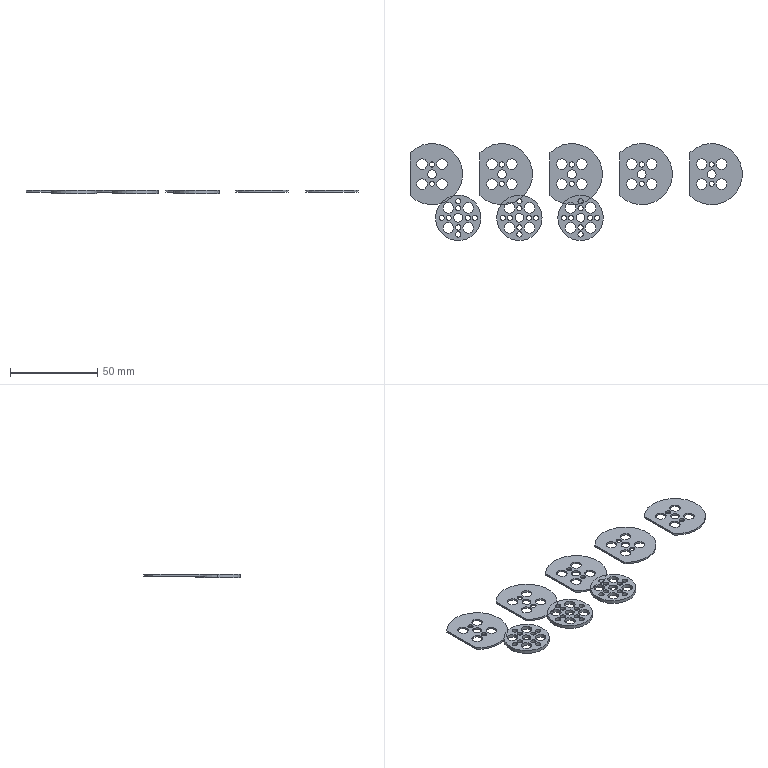CAM job | Mastercam | mm | 7 operations | part box 190.1 x 55.5 x 2
1. Drill/Counterbore | 5 - 4 倒角刀
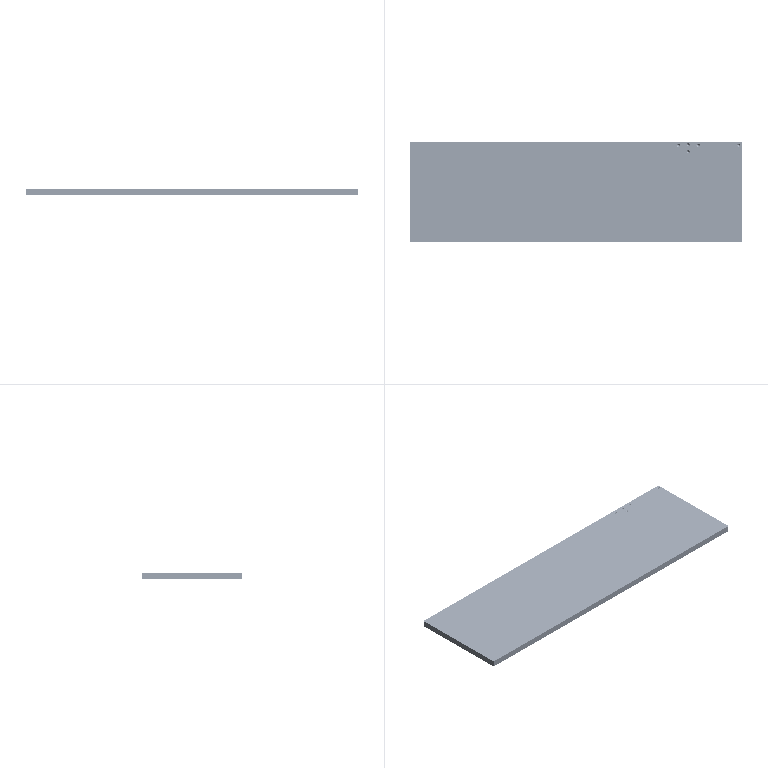2. Contour (Ramp) | 2 - 2 平铣刀
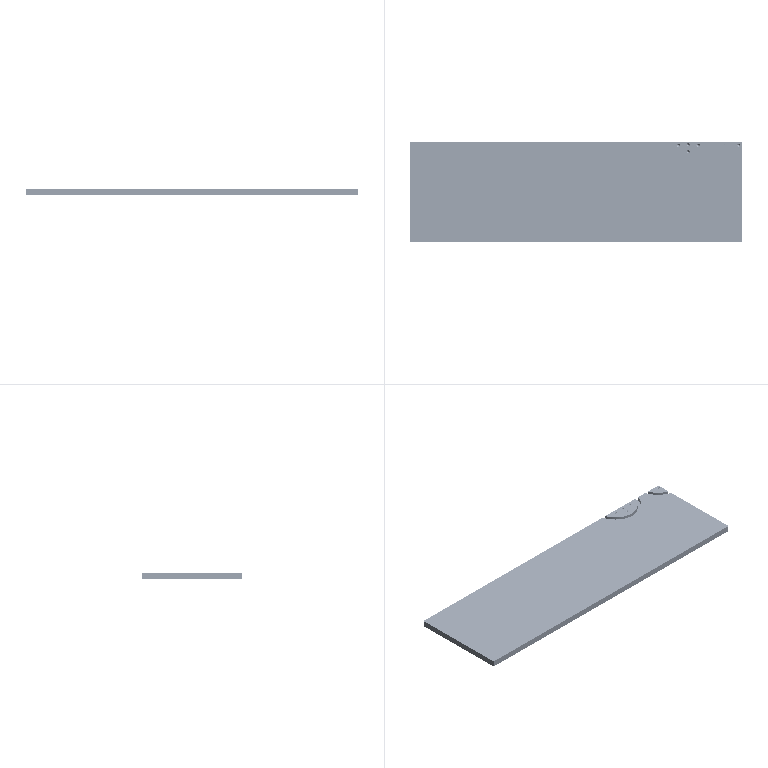3. Contour (2D chamfer) | 5 - 4 倒角刀
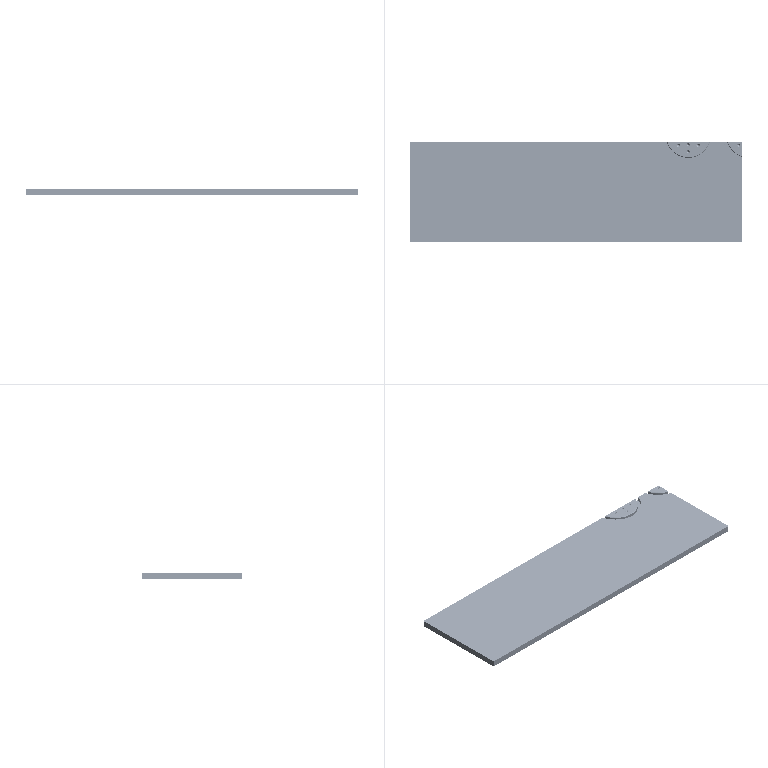4. Contour (Ramp) | 3 - 3 平铣刀
5. Contour (Ramp) | 2 - 2 平铣刀
6. Contour (Ramp) | 2 - 2 平铣刀
7. Contour (2D chamfer) | 7 - 6 倒角刀